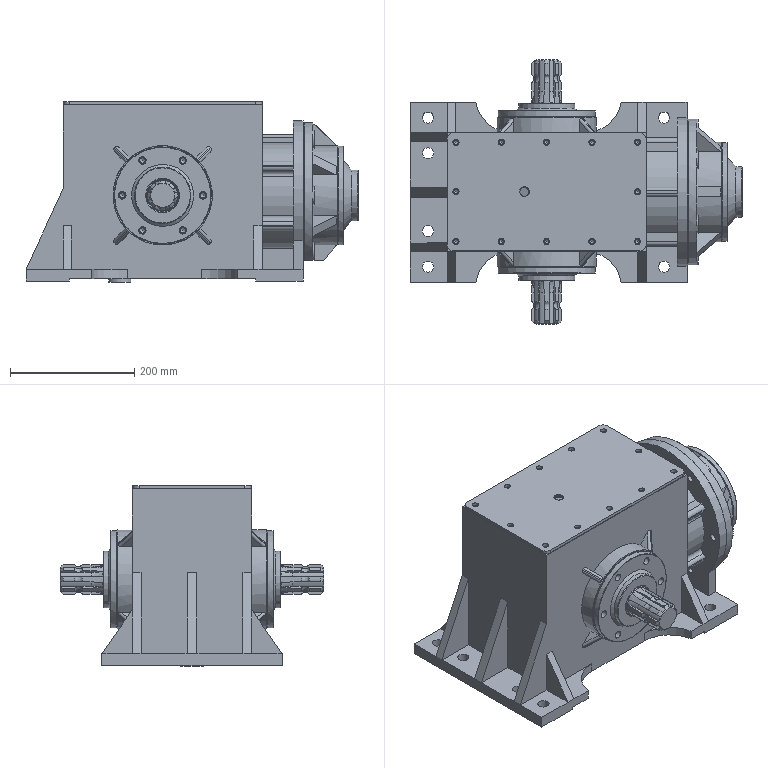Assembly | NX | mm | 17 component files | 18 solids | 712 faces | box 534.5 x 425 x 291 mm | volume 8338403 mm3 | cylinder 278 | plane 243 | cone 157 | torus 32 | spline 2 | commonest cylinder face diameters 12 x30 8.5 x20 14 x19 48 x18 8 x16 40.5 x16 10 x14 6.8 x12
Bill of materials:
unnamed part 1 | 1 |  | Plain thin-walled cylindrical tube or sleeve, open at both ends, with a uniform round bore.
unnamed part 2 | 2 |  | Thin flat annular plate (gasket- or shim-like) with a large central opening, six through-holes on a bolt circle, and one straight cut edge across the bottom of the outer circle.
unnamed part 3 | 1 |  | Thin flat annular plate with a central opening, six through-holes on a bolt circle, and one straight cut edge on the outer circle. The central opening looks smaller relative to the outside diameter than in unnamed part 2.
unnamed part 4 | 1 |  | Housing-like body: a rectangular box with an open top framed by a flat rim with a row of small holes. Two opposite side walls carry raised round bosses or flanges with large bores, bolt-hole circles and triangular ribs. Ribbed mounting feet at the base have through-holes, and the base has arched cutouts.
unnamed part 5 | 1 |  | Round flange-type part: a flat circular disc with six through-holes on a bolt circle, a conical transition up to a smaller cylindrical spigot or hub, and a central through-bore. A thin raised step is also visible on the back face.
unnamed part 6 | 1 |  | Thin flat annular ring with a large central opening and six evenly spaced through-holes. The outer edge is fully circular with no flat.
unnamed part 7 | 1 |  | Stepped cylindrical shaft. Its central larger-diameter section carries raised longitudinal ridges (spline- or key-like). Both ends have splined sections with longitudinal teeth and a circumferential groove near each end.
unnamed part 8 | 4 |  | Plain flat washer-like ring: a rectangular-section annulus with a moderate radial width and modest axial thickness.
unnamed part 9 | 1 |  | Flanged sleeve or hub: a long plain cylindrical barrel attached to a large circular flange. The flange carries several bolt holes on an outer circle and smaller holes on an inner circle. Triangular gusset ribs link it to a short raised collar around the central bore.
unnamed part 10 | 1 |  | Thick plain ring or spacer with a rectangular cross-section. It is axially thicker relative to its diameter than the thin rings.
unnamed part 11 | 2 |  | Round flange-type plate with a central through-bore and six evenly spaced through-holes on a bolt circle. A raised stepped spigot sits on one face, a shallower step on the other, and concentric grooves or steps are visible around the bore.
unnamed part 12 | 1 |  | Thin flat rectangular plate with rounded corners and twelve through-holes around the edge (five along each long side, one centred on each short side). One off-centre hole appears threaded or recessed.
Mates:
1. touch align | oil_seal_72x50x8 2 face | oil_seal_72x50x8 3 face
2. touch align | oil_seal_72x50x8 2 face | oil_seal_72x50x8 3 face
3. touch align | oil_seal_72x50x8 4 face | oil_seal_72x50x8 1 face
4. touch align | oil_seal_72x50x8 1 face | oil_seal_72x50x8 4 face
5. touch align | oil_seal_72x50x8 4 face | side_end_cover 1 face
6. touch align | oil_seal_72x50x8 4 face | side_end_cover 1 face
7. touch align | oil_seal_72x50x8 2 face | side_end_cover 2 face
8. touch align | oil_seal_72x50x8 2 face | side_end_cover 2 face
9. touch align | T1_gasket 2 face | side_end_cover 2 face
10. touch align | T1_gasket 2 face | side_end_cover 2 face
11. touch align | T1_gasket 2 face | side_end_cover 2 face
12. touch align | T1_gasket 1 face | side_end_cover 1 face
13. touch align | T1_gasket 1 face | side_end_cover 1 face
14. touch align | T1_gasket 1 face | side_end_cover 1 face
15. touch align | T1_gasket 1 face | housing_shell 1 face
16. touch align | T1_gasket 2 face | housing_shell 1 face
17. touch align | T1_gasket 2 face | housing_shell 1 face
18. touch align | T1_gasket 1 face | housing_shell 1 face
19. touch align | side_end_cover 1 face | housing_shell 1 face
20. touch align | side_end_cover 2 face | housing_shell 1 face
21. fix | housing_shell 1 component
22. touch align | spacer_sleeve 1 face | shaft 1 face
23. center | shaft 1 face | shaft 1 face | housing_shell 1 face | housing_shell 1 face
24. touch align | spacer_sleeve 1 face | housing_shell 1 face
25. touch align | T2_gasket 1 face | housing_shell 1 face
26. touch align | T2_gasket 1 face | housing_shell 1 face
27. touch align | T2_gasket 1 face | housing_shell 1 face
28. touch align | front_bearing_sleeve 1 face | housing_shell 1 face
29. distance | front_bearing_sleeve 1 face | T2_gasket 1 face
30. touch align | front_bearing_sleeve 1 face | housing_shell 1 face
31. touch align | front_bearing_sleeve 1 face | housing_shell 1 face
32. touch align | T1_gasket_2 1 face | front_bearing_sleeve 1 face
33. touch align | T1_gasket_2 1 face | front_bearing_sleeve 1 face
34. touch align | T1_gasket_2 1 face | front_bearing_sleeve 1 face
35. touch align | oil_seal_72x50x12 1 face | front_end_cover 1 face
36. touch align | front_end_cover 1 face | oil_seal_72x50x12 1 face
37. touch align | front_end_cover 1 face | front_bearing_sleeve 1 face
38. touch align | front_end_cover 1 face | front_bearing_sleeve 1 face
39. touch align | front_end_cover 1 face | T1_gasket_2 1 face
40. touch align | T5_cover_plate 1 face | housing_shell 1 face
41. touch align | T5_cover_plate 1 face | housing_shell 1 face
42. touch align | T5_cover_plate 1 face | housing_shell 1 face